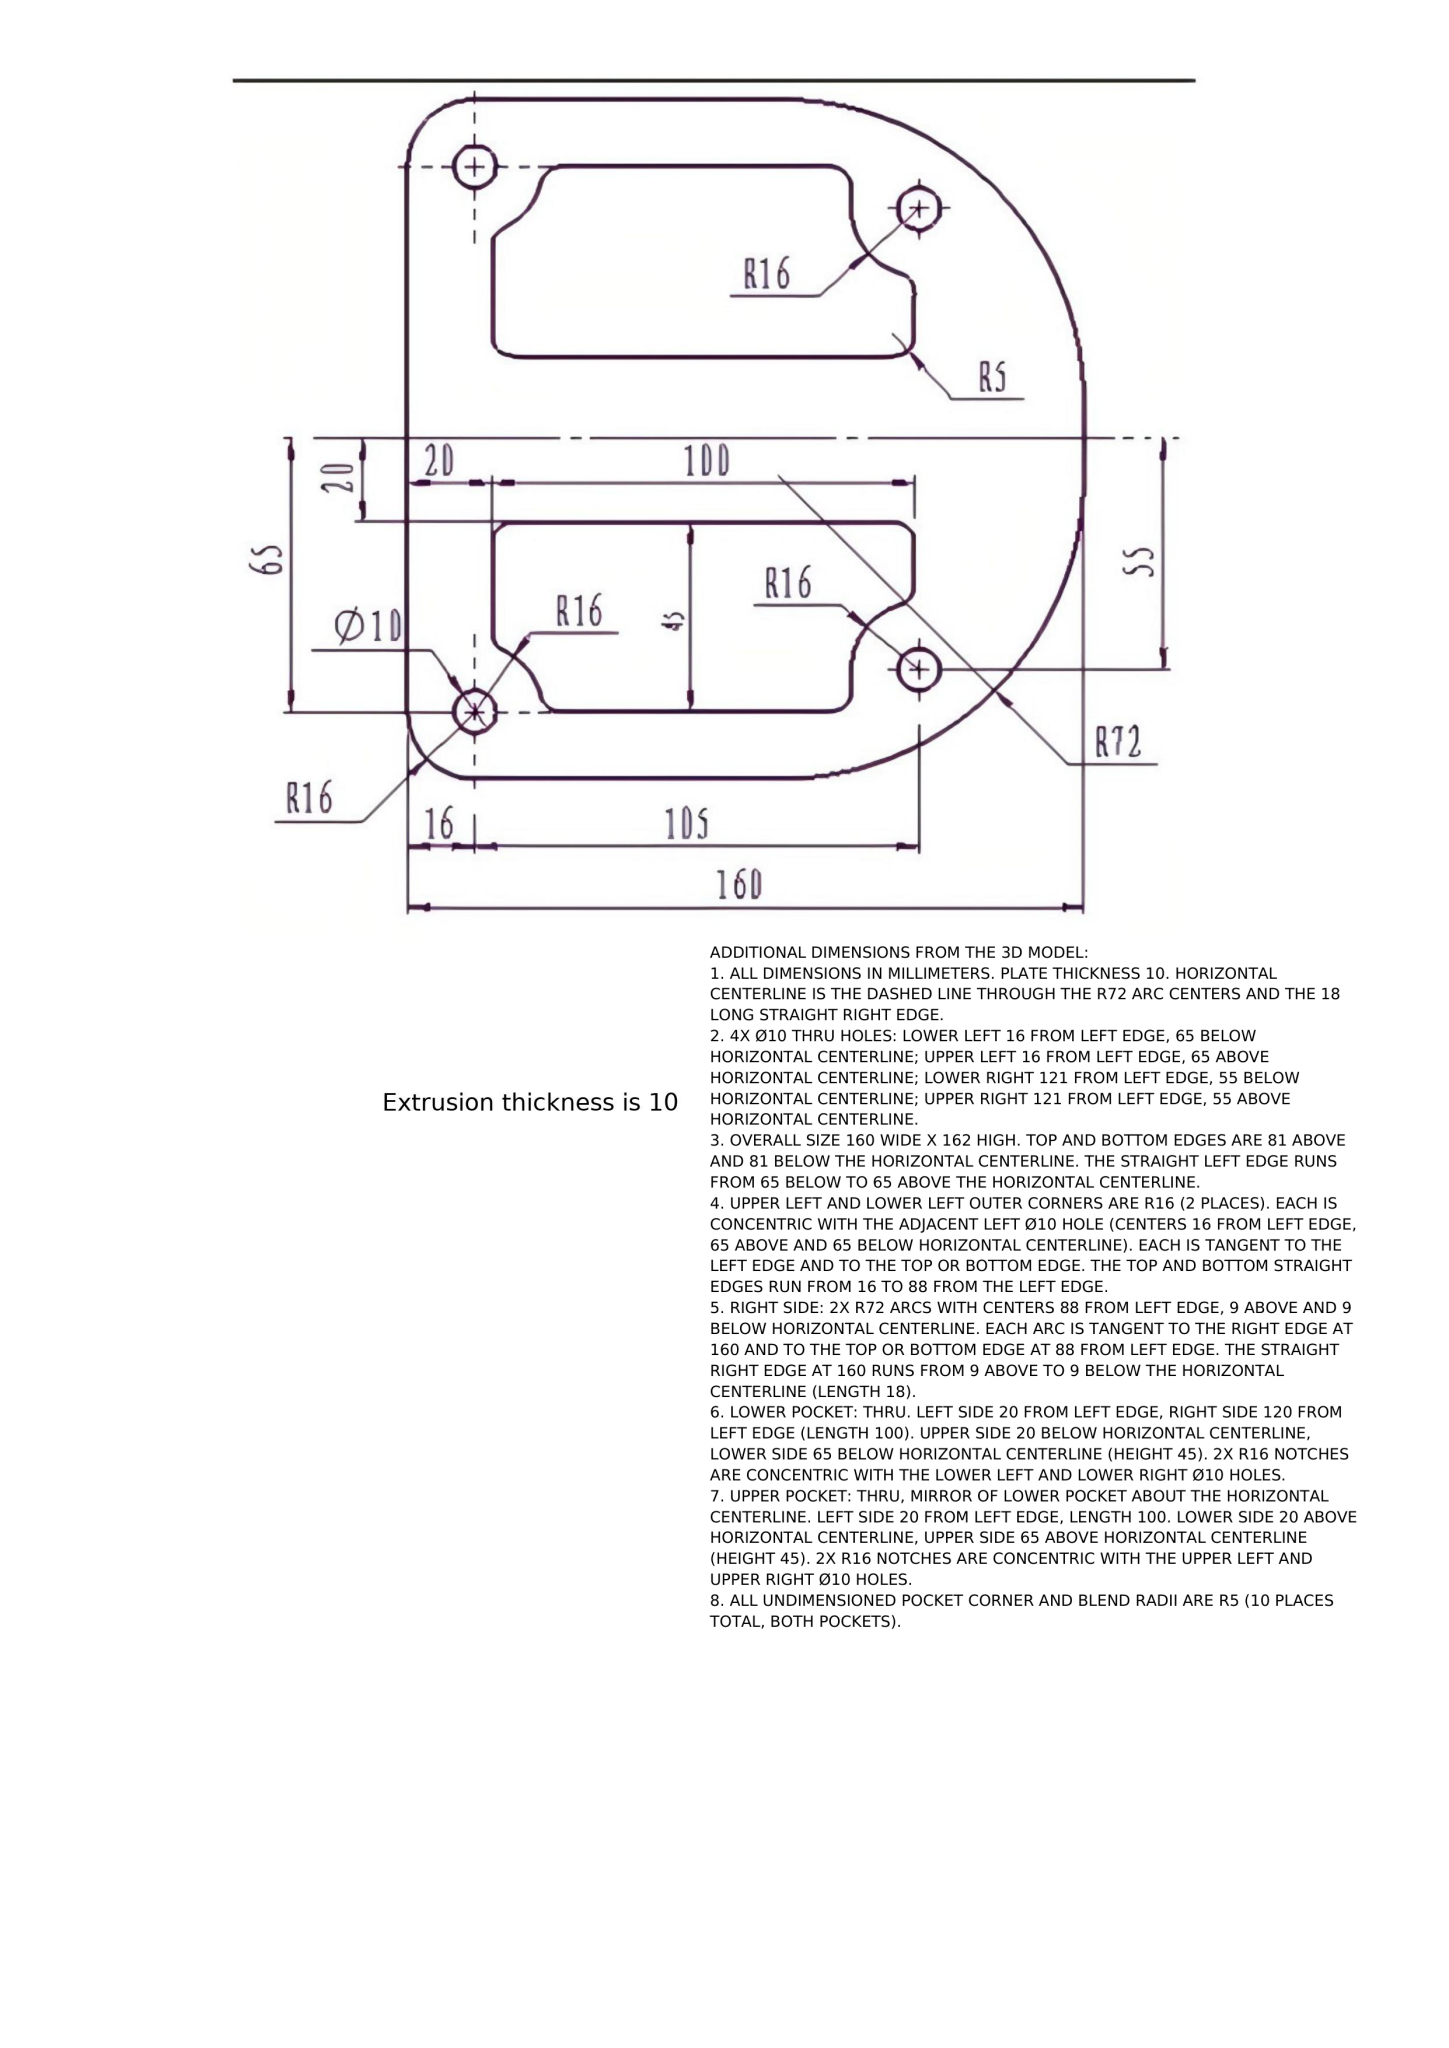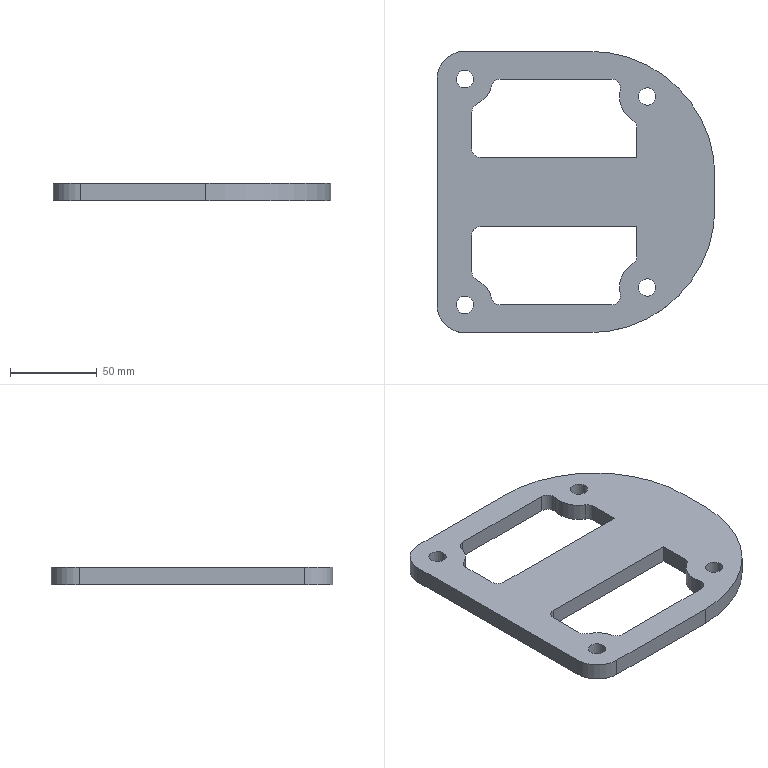Part | NX | mm | 1 solid | 36 faces | box 160 x 162 x 10 mm | volume 154382 mm3 | cylinder 22 | plane 14 | commonest cylinder face diameters 10 x14 32 x6 144 x2